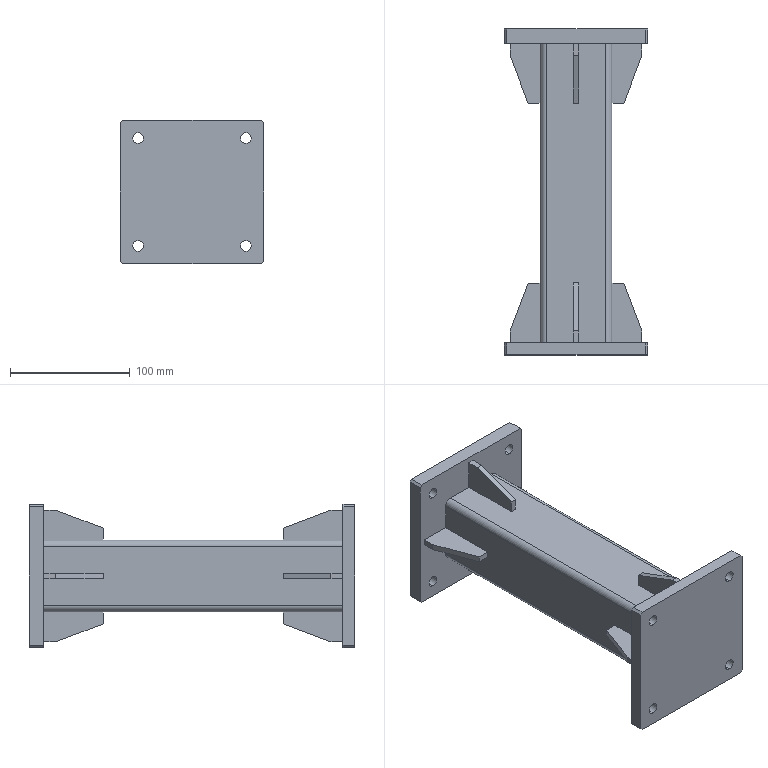Component | SolidWorks | 001-1 | 11 solids | 110 faces | volume 515004 mm3 | plane 86 | cylinder 24 | commonest cylinder face diameters 9 x16 10.8 x4 4.8 x4 | material Q235B